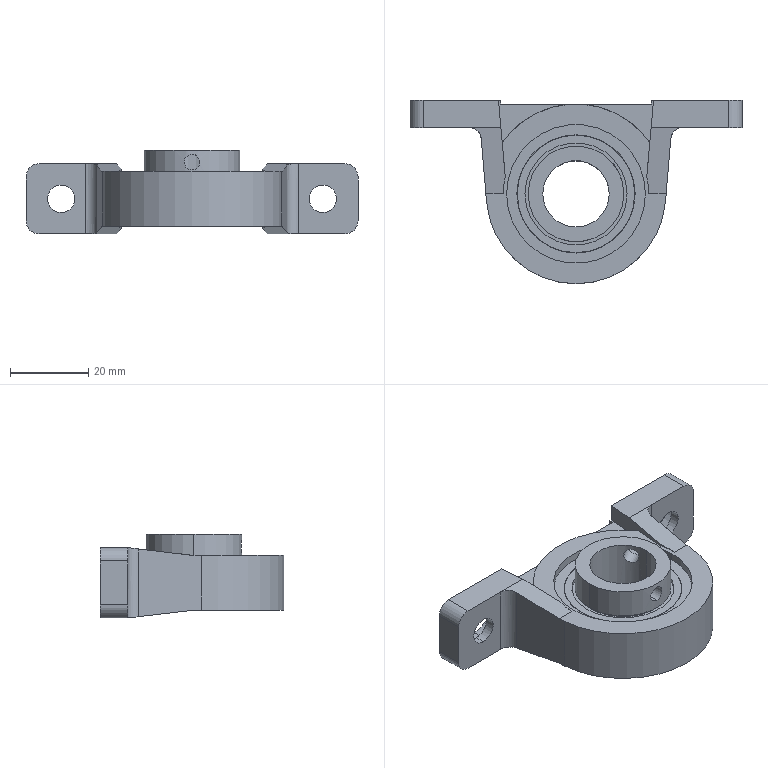Component | SolidWorks | PBT17-2-2_PBT17x-2-1 | 1 solid | 86 faces | volume 25430 mm3 | plane 43 | cylinder 37 | torus 6 | commonest cylinder face diameters 4 x4 7 x4 35.5 x4 37.275 x4 6.8 x4 12 x4 46 x3 26.167 x2